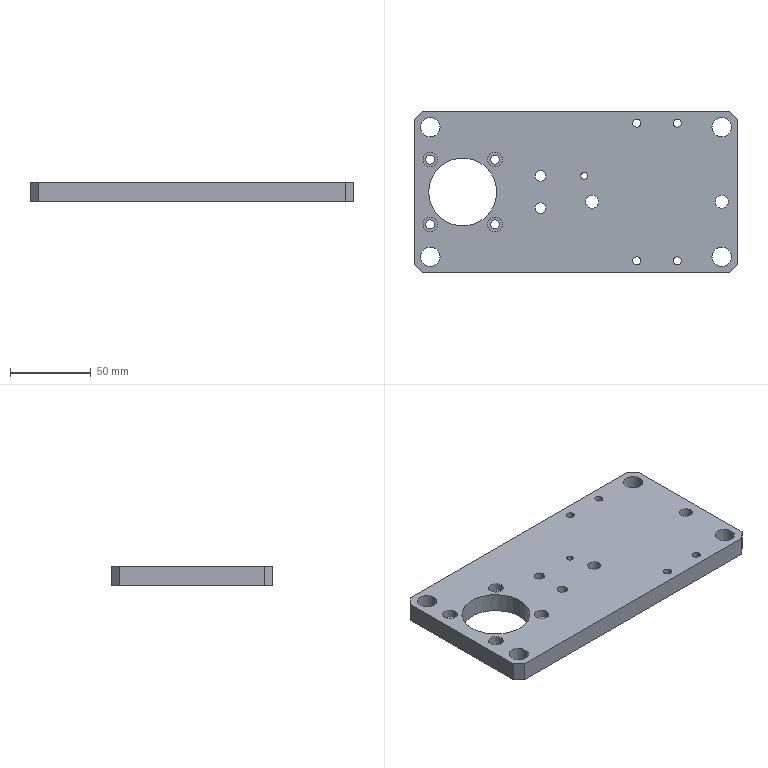Component | SolidWorks | YX-04-103GluePaperFeedingBottomPlate-1 | 1 solid | 74 faces | volume 211330 mm3 | cylinder 48 | plane 16 | cone 10 | commonest cylinder face diameters 12 x12 9 x8 5.5 x8 5 x8 6.5 x4 8 x4 42 x2 4.2 x2 | material 45#Steel